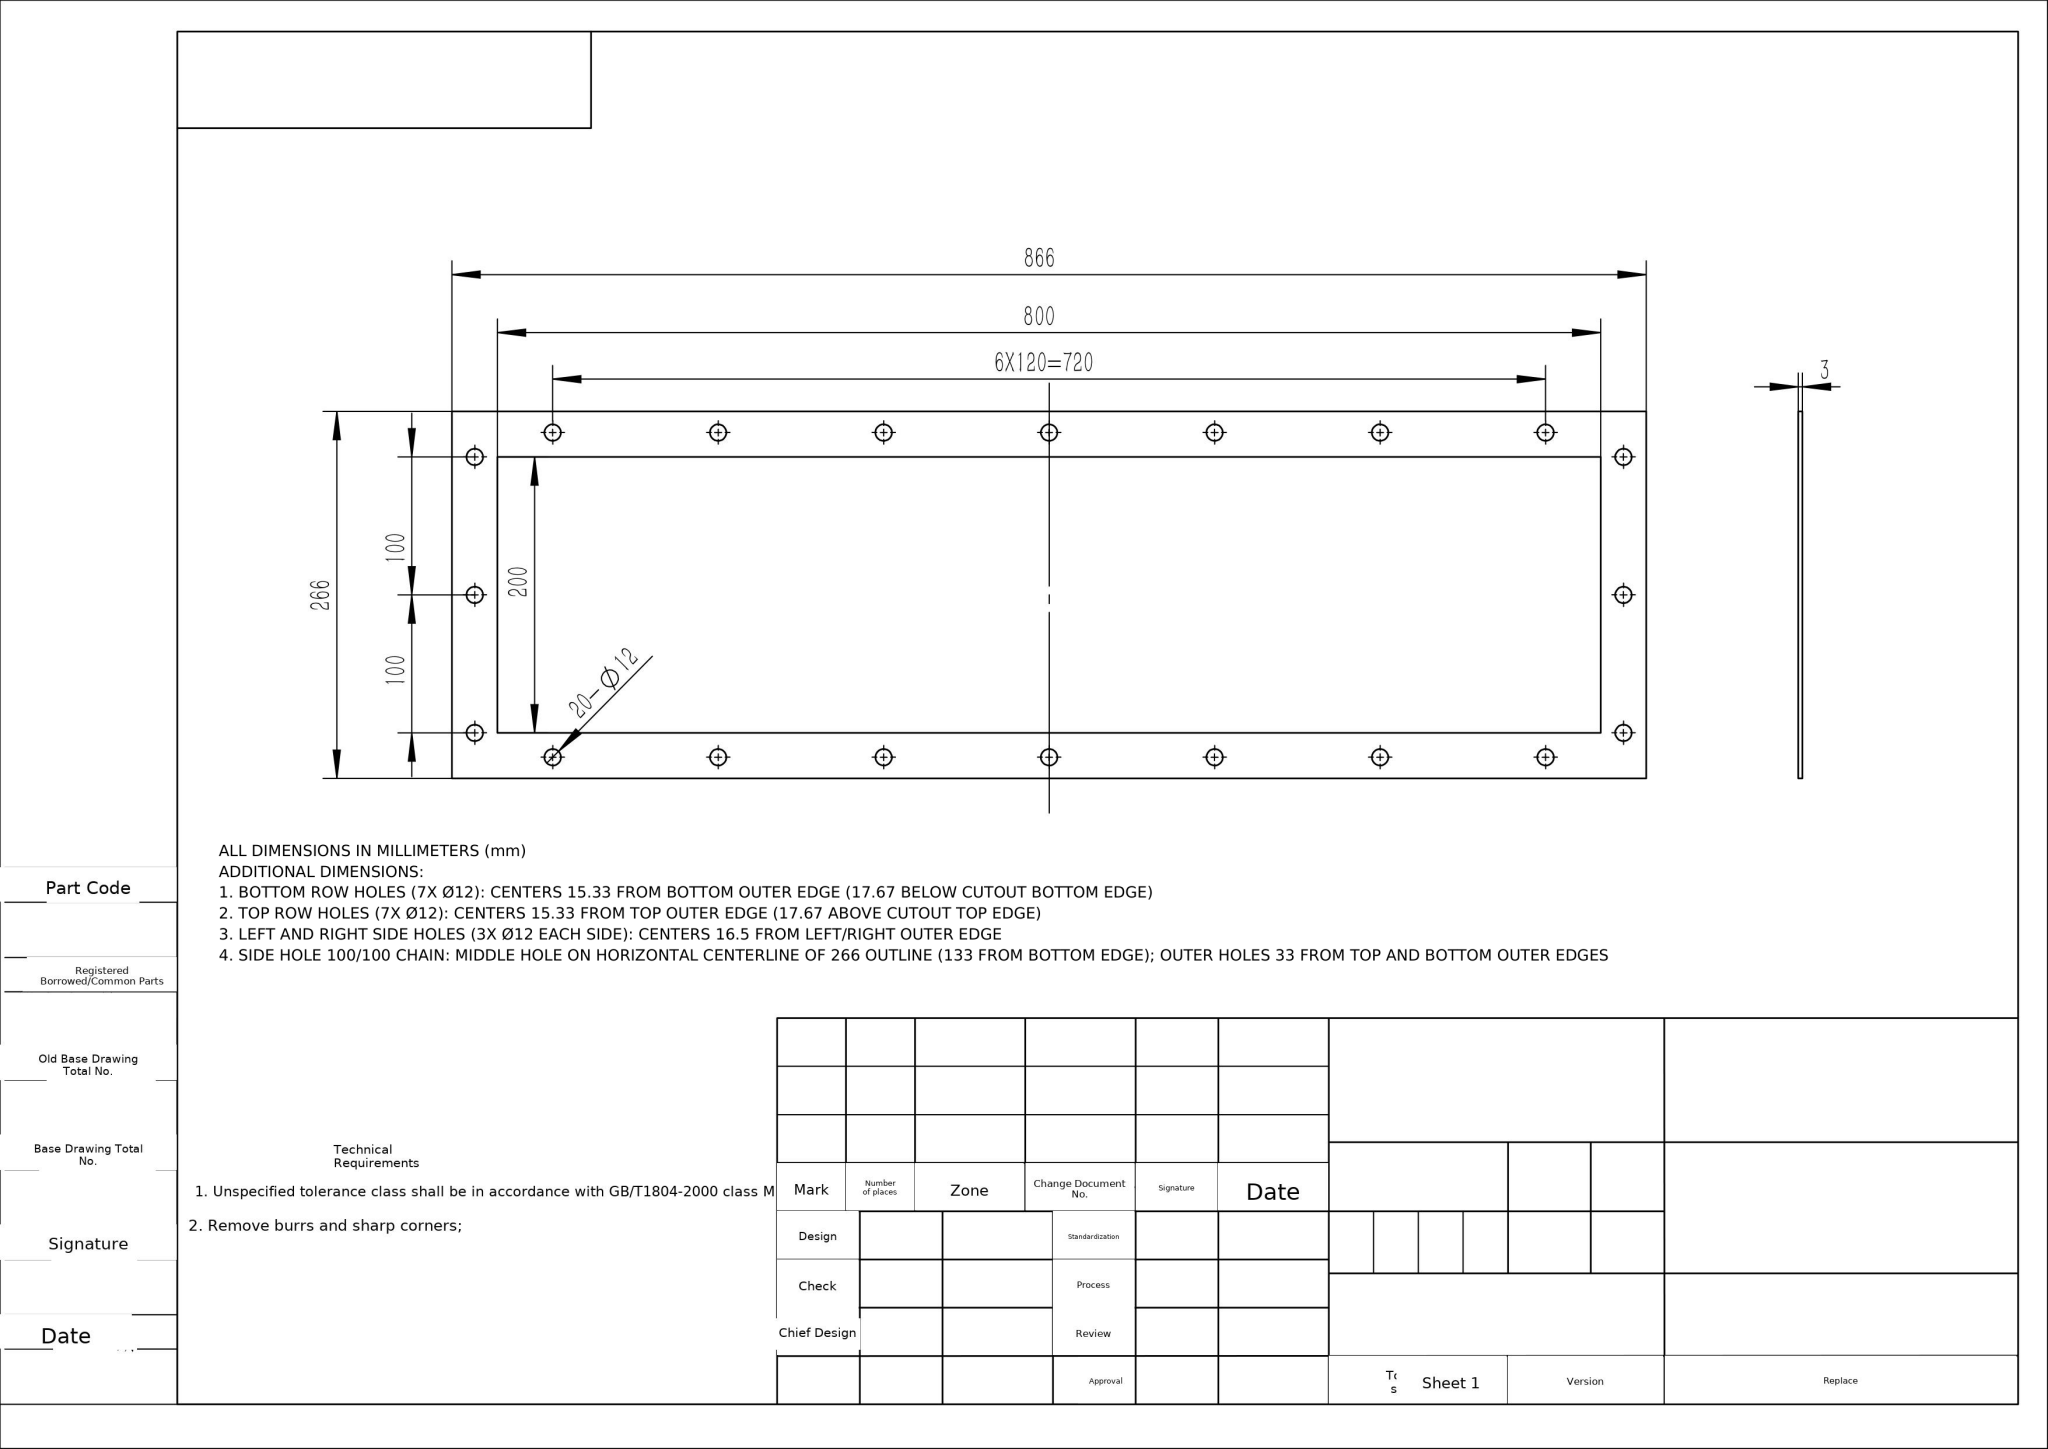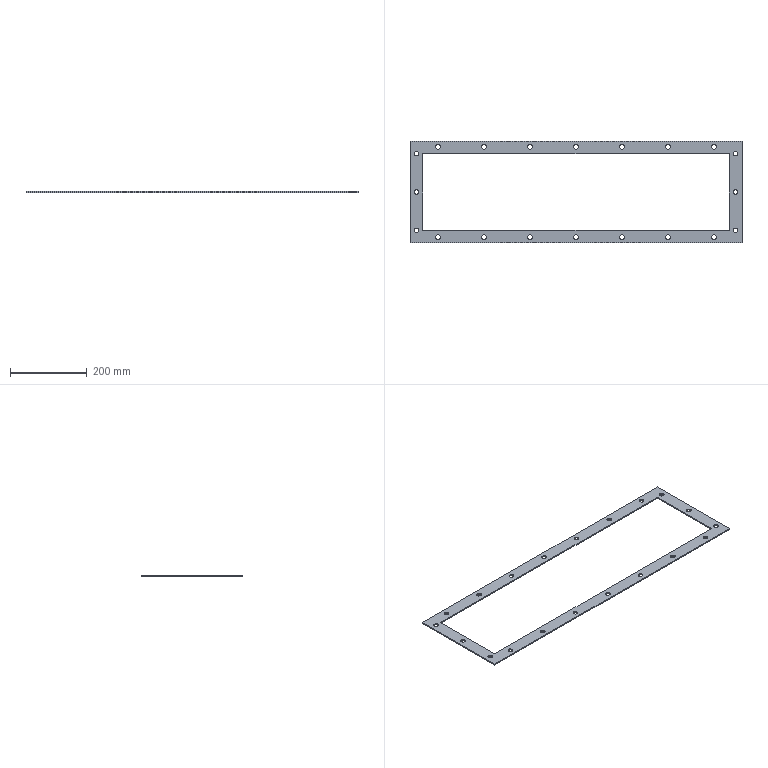Part | NX | mm | 1 solid | 50 faces | box 866 x 266 x 3 mm | volume 204282 mm3 | cylinder 40 | plane 10 | commonest cylinder face diameters 12 x40